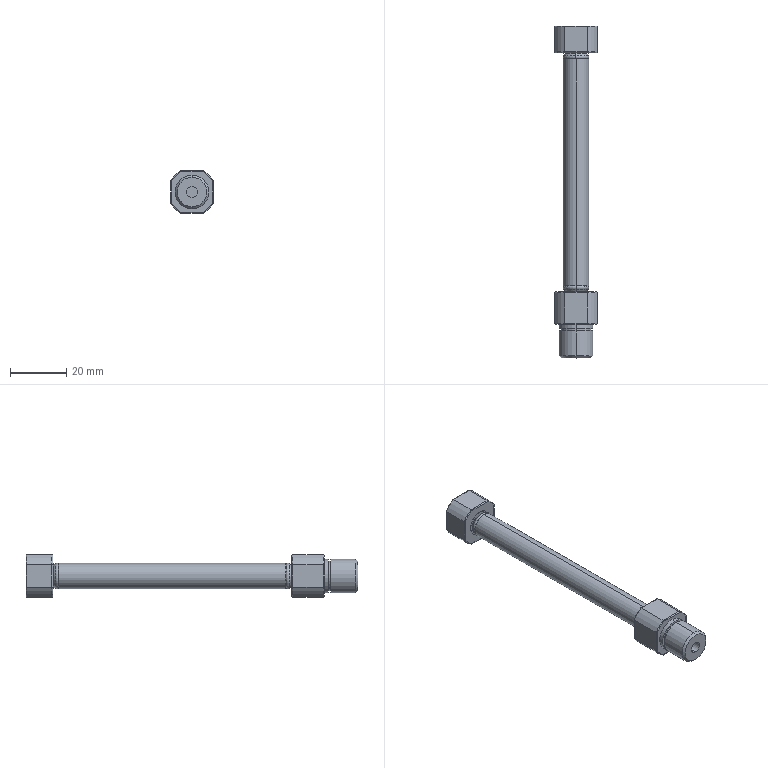Component | SolidWorks | MI-8x60-S-U-M-2(0)-1_MI 8x60-S-U_c-1 | 1 solid | 101 faces | box 15 x 118 x 15 mm | volume 7196 mm3 | cylinder 44 | plane 23 | torus 20 | cone 14 | commonest cylinder face diameters 0.6 x16 17 x8 4.134 x4 9.2 x4 12 x4 7.6 x2 4 x2 9 x2
build123d program:
from build123d import *

# Parameters (mm, degrees)
SKETCH3_W                = 30
SKETCH3_H                = 30
SKETCH3_W_2              = 15
SKETCH3_H_2              = 15
CUT_EXTRUDE1_DEPTH       = 11.5
SKETCH4_W                = 30
SKETCH4_H                = 30
SKETCH4_W_2              = 15
SKETCH4_H_2              = 15
CUT_EXTRUDE2_DEPTH       = 9.5
CUT_EXTRUDE3_DEPTH       = 7.5
CUT_EXTRUDE3_DEPTH_BACK  = 7.5
CUT_EXTRUDE4_DEPTH       = 7.5
CUT_EXTRUDE4_DEPTH_BACK  = 7.5
CUT_EXTRUDE5_DEPTH       = 7.5
CUT_EXTRUDE5_DEPTH_BACK  = 7.5
CUT_EXTRUDE6_DEPTH       = 7.5
CUT_EXTRUDE6_DEPTH_BACK  = 7.5
CUT_EXTRUDE7_DEPTH       = 7.5
CUT_EXTRUDE7_DEPTH_BACK  = 7.5
CUT_EXTRUDE8_DEPTH       = 7.5
CUT_EXTRUDE8_DEPTH_BACK  = 7.5
CUT_EXTRUDE9_DEPTH       = 7.5
CUT_EXTRUDE9_DEPTH_BACK  = 7.5
CUT_EXTRUDE10_DEPTH      = 7.5
CUT_EXTRUDE10_DEPTH_BACK = 7.5
CUT_EXTRUDE11_DEPTH      = 7.5
CUT_EXTRUDE11_DEPTH_BACK = 7.5
CUT_EXTRUDE12_DEPTH      = 7.5
CUT_EXTRUDE12_DEPTH_BACK = 7.5
CUT_EXTRUDE13_DEPTH      = 7.5
CUT_EXTRUDE13_DEPTH_BACK = 7.5
CUT_EXTRUDE14_DEPTH      = 7.5
CUT_EXTRUDE14_DEPTH_BACK = 7.5
CUT_EXTRUDE15_DEPTH      = 7.5
CUT_EXTRUDE15_DEPTH_BACK = 7.5
CUT_EXTRUDE16_DEPTH      = 7.5
CUT_EXTRUDE16_DEPTH_BACK = 7.5
CUT_EXTRUDE17_DEPTH      = 7.5
CUT_EXTRUDE17_DEPTH_BACK = 7.5
CUT_EXTRUDE18_DEPTH      = 7.5
CUT_EXTRUDE18_DEPTH_BACK = 7.5
HOLE1_D                  = 4.134
HOLE1_DEPTH              = 5
HOLE1_CSINK_D            = 5
HOLE1_CSINK_ANGLE        = 90
HOLE2_D                  = 4.134
HOLE2_DEPTH              = 5
HOLE2_CSINK_D            = 5
HOLE2_CSINK_ANGLE        = 90


with BuildPart() as part:
    # Sketch1 → Revolve1 (revolve)
    with BuildSketch(Plane.XY, mode=Mode.PRIVATE) as revolve1_sk:
        Polygon((-12, 0), (-12, 5.233), (-11.233, 6), (-2.4, 6), (-2.4, 5.25), (-1.5, 5.25), (-1.5, 6), (0, 6), (0, 0), align=None)
    revolve(revolve1_sk.sketch.rotate(Axis((0, 0, 0), (-1, 0, 0)), 270), axis=Axis((0, 0, 0), (-1, 0, 0)))

    # Sketch2 → Revolve2 (revolve)
    with BuildSketch(Plane.XY, mode=Mode.PRIVATE) as revolve2_sk:
        with BuildLine():
            Line((0, 0), (0, 8.2))
            ThreePointArc((0, 8.2), (0.08787, 8.412), (0.3, 8.5))
            Line((0.3, 8.5), (11.2, 8.5))
            ThreePointArc((11.2, 8.5), (11.412, 8.412), (11.5, 8.2))
            Line((11.5, 8.2), (11.5, 4.6))
            Line((11.5, 4.6), (11.6, 4.6))
            Line((11.6, 4.6), (11.6, 3.8))
            Line((11.6, 3.8), (12.5, 4.4))
            ThreePointArc((12.5, 4.4), (13, 4.6), (13.5, 4.4))
            Line((13.5, 4.4), (13.5, 4.3))
            Line((13.5, 4.3), (13.7, 4.5))
            Line((13.7, 4.5), (94.3, 4.5))
            Line((94.3, 4.5), (94.5, 4.3))
            Line((94.5, 4.3), (94.5, 4.4))
            ThreePointArc((94.5, 4.4), (95, 4.6), (95.5, 4.4))
            Line((95.5, 4.4), (96.4, 3.8))
            Line((96.4, 3.8), (96.4, 4.6))
            Line((96.4, 4.6), (96.5, 4.6))
            Line((96.5, 4.6), (96.5, 8.2))
            ThreePointArc((96.5, 8.2), (96.588, 8.412), (96.8, 8.5))
            Line((96.8, 8.5), (105.7, 8.5))
            ThreePointArc((105.7, 8.5), (105.912, 8.412), (106, 8.2))
            Line((106, 8.2), (106, 0))
            Line((106, 0), (0, 0))
        make_face()
    revolve(revolve2_sk.sketch.rotate(Axis((106, 0, 0), (-1, 0, 0)), 270), axis=Axis((106, 0, 0), (-1, 0, 0)))

    # Sketch3 → Cut-Extrude1 (cut)
    with BuildSketch(Plane(origin=(0, 0, 0), x_dir=(0, 0, -1), z_dir=(1, 0, 0))):
        Rectangle(SKETCH3_W, SKETCH3_H)
        Rectangle(SKETCH3_W_2, SKETCH3_H_2, mode=Mode.SUBTRACT)
    extrude(amount=CUT_EXTRUDE1_DEPTH, mode=Mode.SUBTRACT)

    # Sketch4 → Cut-Extrude2 (cut)
    with BuildSketch(Plane(origin=(106, 0, 0), x_dir=(0, 0, -1), z_dir=(1, 0, 0))):
        Rectangle(SKETCH4_W, SKETCH4_H)
        Rectangle(SKETCH4_W_2, SKETCH4_H_2, mode=Mode.SUBTRACT)
    extrude(amount=-CUT_EXTRUDE2_DEPTH, mode=Mode.SUBTRACT)

    # Sketch5 → Cut-Extrude3 (cut, two sides: drawn at the far end of the back side and taken through both)
    with BuildSketch(Plane.XY.offset(-CUT_EXTRUDE3_DEPTH_BACK)):
        with BuildLine():
            Line((0, 7.5), (0, 7.2))
            ThreePointArc((0, 7.2), (0.08787, 7.412), (0.3, 7.5))
            Line((0.3, 7.5), (0, 7.5))
        make_face()
    extrude(amount=CUT_EXTRUDE3_DEPTH + CUT_EXTRUDE3_DEPTH_BACK, mode=Mode.SUBTRACT)

    # Sketch6 → Cut-Extrude4 (cut, two sides: drawn at the far end of the back side and taken through both)
    with BuildSketch(Plane.XY.offset(-CUT_EXTRUDE4_DEPTH_BACK)):
        with BuildLine():
            Line((0, -7.5), (0.3, -7.5))
            ThreePointArc((0.3, -7.5), (0.08787, -7.412), (0, -7.2))
            Line((0, -7.2), (0, -7.5))
        make_face()
    extrude(amount=CUT_EXTRUDE4_DEPTH + CUT_EXTRUDE4_DEPTH_BACK, mode=Mode.SUBTRACT)

    # Sketch7 → Cut-Extrude5 (cut, two sides: drawn at the far end of the back side and taken through both)
    with BuildSketch(Plane(origin=(0, 0, 0), x_dir=(1, 0, 0), z_dir=(0, 1, 0)).offset(-CUT_EXTRUDE5_DEPTH_BACK)):
        with BuildLine():
            Line((0, 7.5), (0, 7.2))
            ThreePointArc((0, 7.2), (0.08787, 7.412), (0.3, 7.5))
            Line((0.3, 7.5), (0, 7.5))
        make_face()
    extrude(amount=CUT_EXTRUDE5_DEPTH + CUT_EXTRUDE5_DEPTH_BACK, mode=Mode.SUBTRACT)

    # Sketch8 → Cut-Extrude6 (cut, two sides: drawn at the far end of the back side and taken through both)
    with BuildSketch(Plane(origin=(0, 0, 0), x_dir=(1, 0, 0), z_dir=(0, 1, 0)).offset(-CUT_EXTRUDE6_DEPTH_BACK)):
        with BuildLine():
            Line((0, -7.5), (0.3, -7.5))
            ThreePointArc((0.3, -7.5), (0.08787, -7.412), (0, -7.2))
            Line((0, -7.2), (0, -7.5))
        make_face()
    extrude(amount=CUT_EXTRUDE6_DEPTH + CUT_EXTRUDE6_DEPTH_BACK, mode=Mode.SUBTRACT)

    # Sketch9 → Cut-Extrude7 (cut, two sides: drawn at the far end of the back side and taken through both)
    with BuildSketch(Plane.XY.offset(-CUT_EXTRUDE7_DEPTH_BACK)):
        with BuildLine():
            Line((11.5, 7.2), (11.5, 7.5))
            Line((11.5, 7.5), (11.2, 7.5))
            ThreePointArc((11.2, 7.5), (11.412, 7.412), (11.5, 7.2))
        make_face()
    extrude(amount=CUT_EXTRUDE7_DEPTH + CUT_EXTRUDE7_DEPTH_BACK, mode=Mode.SUBTRACT)

    # Sketch10 → Cut-Extrude8 (cut, two sides: drawn at the far end of the back side and taken through both)
    with BuildSketch(Plane.XY.offset(-CUT_EXTRUDE8_DEPTH_BACK)):
        with BuildLine():
            Line((11.2, -7.5), (11.5, -7.5))
            Line((11.5, -7.5), (11.5, -7.2))
            ThreePointArc((11.5, -7.2), (11.412, -7.412), (11.2, -7.5))
        make_face()
    extrude(amount=CUT_EXTRUDE8_DEPTH + CUT_EXTRUDE8_DEPTH_BACK, mode=Mode.SUBTRACT)

    # Sketch11 → Cut-Extrude9 (cut, two sides: drawn at the far end of the back side and taken through both)
    with BuildSketch(Plane(origin=(0, 0, 0), x_dir=(1, 0, 0), z_dir=(0, 1, 0)).offset(-CUT_EXTRUDE9_DEPTH_BACK)):
        with BuildLine():
            Line((11.5, 7.2), (11.5, 7.5))
            Line((11.5, 7.5), (11.2, 7.5))
            ThreePointArc((11.2, 7.5), (11.412, 7.412), (11.5, 7.2))
        make_face()
    extrude(amount=CUT_EXTRUDE9_DEPTH + CUT_EXTRUDE9_DEPTH_BACK, mode=Mode.SUBTRACT)

    # Sketch12 → Cut-Extrude10 (cut, two sides: drawn at the far end of the back side and taken through both)
    with BuildSketch(Plane(origin=(0, 0, 0), x_dir=(1, 0, 0), z_dir=(0, 1, 0)).offset(-CUT_EXTRUDE10_DEPTH_BACK)):
        with BuildLine():
            Line((11.2, -7.5), (11.5, -7.5))
            Line((11.5, -7.5), (11.5, -7.2))
            ThreePointArc((11.5, -7.2), (11.412, -7.412), (11.2, -7.5))
        make_face()
    extrude(amount=CUT_EXTRUDE10_DEPTH + CUT_EXTRUDE10_DEPTH_BACK, mode=Mode.SUBTRACT)

    # Sketch13 → Cut-Extrude11 (cut, two sides: drawn at the far end of the back side and taken through both)
    with BuildSketch(Plane.XY.offset(-CUT_EXTRUDE11_DEPTH_BACK)):
        with BuildLine():
            Line((106, 7.2), (106, 7.5))
            Line((106, 7.5), (105.7, 7.5))
            ThreePointArc((105.7, 7.5), (105.912, 7.412), (106, 7.2))
        make_face()
    extrude(amount=CUT_EXTRUDE11_DEPTH + CUT_EXTRUDE11_DEPTH_BACK, mode=Mode.SUBTRACT)

    # Sketch14 → Cut-Extrude12 (cut, two sides: drawn at the far end of the back side and taken through both)
    with BuildSketch(Plane.XY.offset(-CUT_EXTRUDE12_DEPTH_BACK)):
        with BuildLine():
            Line((105.7, -7.5), (106, -7.5))
            Line((106, -7.5), (106, -7.2))
            ThreePointArc((106, -7.2), (105.912, -7.412), (105.7, -7.5))
        make_face()
    extrude(amount=CUT_EXTRUDE12_DEPTH + CUT_EXTRUDE12_DEPTH_BACK, mode=Mode.SUBTRACT)

    # Sketch15 → Cut-Extrude13 (cut, two sides: drawn at the far end of the back side and taken through both)
    with BuildSketch(Plane(origin=(0, 0, 0), x_dir=(1, 0, 0), z_dir=(0, 1, 0)).offset(-CUT_EXTRUDE13_DEPTH_BACK)):
        with BuildLine():
            Line((106, 7.2), (106, 7.5))
            Line((106, 7.5), (105.7, 7.5))
            ThreePointArc((105.7, 7.5), (105.912, 7.412), (106, 7.2))
        make_face()
    extrude(amount=CUT_EXTRUDE13_DEPTH + CUT_EXTRUDE13_DEPTH_BACK, mode=Mode.SUBTRACT)

    # Sketch16 → Cut-Extrude14 (cut, two sides: drawn at the far end of the back side and taken through both)
    with BuildSketch(Plane(origin=(0, 0, 0), x_dir=(1, 0, 0), z_dir=(0, 1, 0)).offset(-CUT_EXTRUDE14_DEPTH_BACK)):
        with BuildLine():
            Line((105.7, -7.5), (106, -7.5))
            Line((106, -7.5), (106, -7.2))
            ThreePointArc((106, -7.2), (105.912, -7.412), (105.7, -7.5))
        make_face()
    extrude(amount=CUT_EXTRUDE14_DEPTH + CUT_EXTRUDE14_DEPTH_BACK, mode=Mode.SUBTRACT)

    # Sketch17 → Cut-Extrude15 (cut, two sides: drawn at the far end of the back side and taken through both)
    with BuildSketch(Plane.XY.offset(-CUT_EXTRUDE15_DEPTH_BACK)):
        with BuildLine():
            Line((96.8, 7.5), (96.5, 7.5))
            Line((96.5, 7.5), (96.5, 7.2))
            ThreePointArc((96.5, 7.2), (96.588, 7.412), (96.8, 7.5))
        make_face()
    extrude(amount=CUT_EXTRUDE15_DEPTH + CUT_EXTRUDE15_DEPTH_BACK, mode=Mode.SUBTRACT)

    # Sketch18 → Cut-Extrude16 (cut, two sides: drawn at the far end of the back side and taken through both)
    with BuildSketch(Plane.XY.offset(-CUT_EXTRUDE16_DEPTH_BACK)):
        with BuildLine():
            Line((96.5, -7.2), (96.5, -7.5))
            Line((96.5, -7.5), (96.8, -7.5))
            ThreePointArc((96.8, -7.5), (96.588, -7.412), (96.5, -7.2))
        make_face()
    extrude(amount=CUT_EXTRUDE16_DEPTH + CUT_EXTRUDE16_DEPTH_BACK, mode=Mode.SUBTRACT)

    # Sketch19 → Cut-Extrude17 (cut, two sides: drawn at the far end of the back side and taken through both)
    with BuildSketch(Plane(origin=(0, 0, 0), x_dir=(1, 0, 0), z_dir=(0, 1, 0)).offset(-CUT_EXTRUDE17_DEPTH_BACK)):
        with BuildLine():
            Line((96.8, 7.5), (96.5, 7.5))
            Line((96.5, 7.5), (96.5, 7.2))
            ThreePointArc((96.5, 7.2), (96.588, 7.412), (96.8, 7.5))
        make_face()
    extrude(amount=CUT_EXTRUDE17_DEPTH + CUT_EXTRUDE17_DEPTH_BACK, mode=Mode.SUBTRACT)

    # Sketch20 → Cut-Extrude18 (cut, two sides: drawn at the far end of the back side and taken through both)
    with BuildSketch(Plane(origin=(0, 0, 0), x_dir=(1, 0, 0), z_dir=(0, 1, 0)).offset(-CUT_EXTRUDE18_DEPTH_BACK)):
        with BuildLine():
            Line((96.5, -7.2), (96.5, -7.5))
            Line((96.5, -7.5), (96.8, -7.5))
            ThreePointArc((96.8, -7.5), (96.588, -7.412), (96.5, -7.2))
        make_face()
    extrude(amount=CUT_EXTRUDE18_DEPTH + CUT_EXTRUDE18_DEPTH_BACK, mode=Mode.SUBTRACT)

    # Hole1
    with Locations(Plane(origin=(0, 7.5, 0), x_dir=(1, 0, 0), z_dir=(0, 1, 0))):
        with Locations((7, 0)):
            CounterSinkHole(HOLE1_D / 2, HOLE1_CSINK_D / 2, depth=HOLE1_DEPTH, counter_sink_angle=HOLE1_CSINK_ANGLE)

    # Hole2
    with Locations(Plane(origin=(0, 7.5, 0), x_dir=(1, 0, 0), z_dir=(0, 1, 0))):
        with Locations((101, 0)):
            CounterSinkHole(HOLE2_D / 2, HOLE2_CSINK_D / 2, depth=HOLE2_DEPTH, counter_sink_angle=HOLE2_CSINK_ANGLE)

    # Sketch25 → Cut-Revolve1 (revolve, cut)
    with BuildSketch(Plane.XY, mode=Mode.PRIVATE) as cut_revolve1_sk:
        Polygon((-17, 0), (-17, 2), (18, 2), (18, 3.8), (91, 3.8), (91, 0), align=None)
    revolve(cut_revolve1_sk.sketch.rotate(Axis((91, 0, 0), (-1, 0, 0)), 270), axis=Axis((91, 0, 0), (-1, 0, 0)), mode=Mode.SUBTRACT)


solid = part.part

# Placed as in the assembly
solid = solid.moved(Location((-44.181, -44.188, -311.979), (180, 0, -90)))